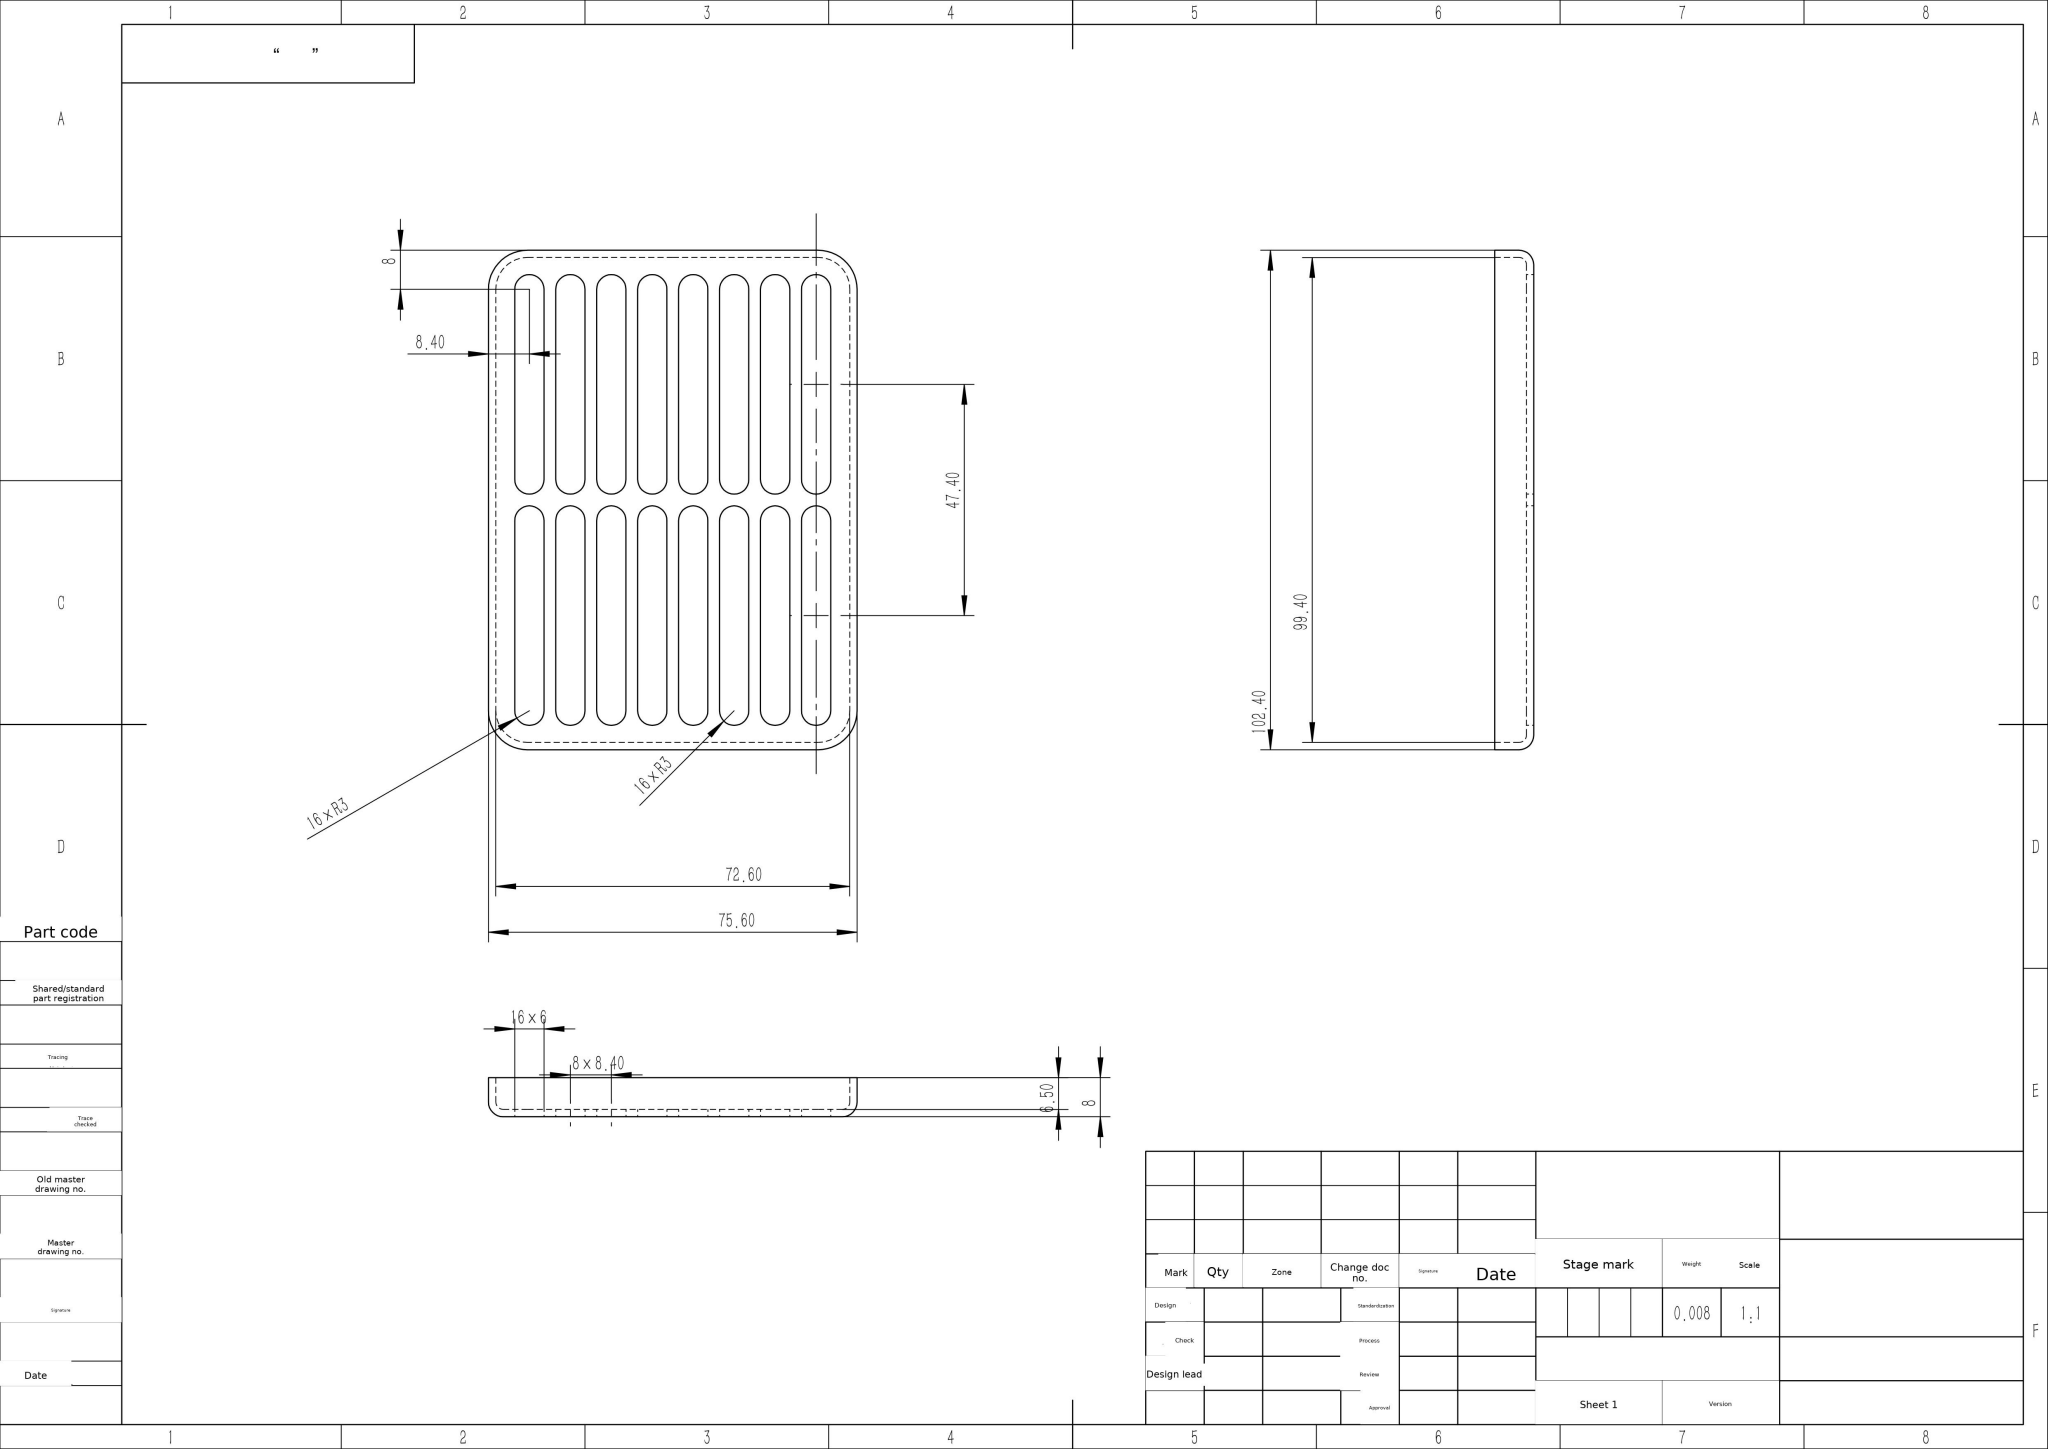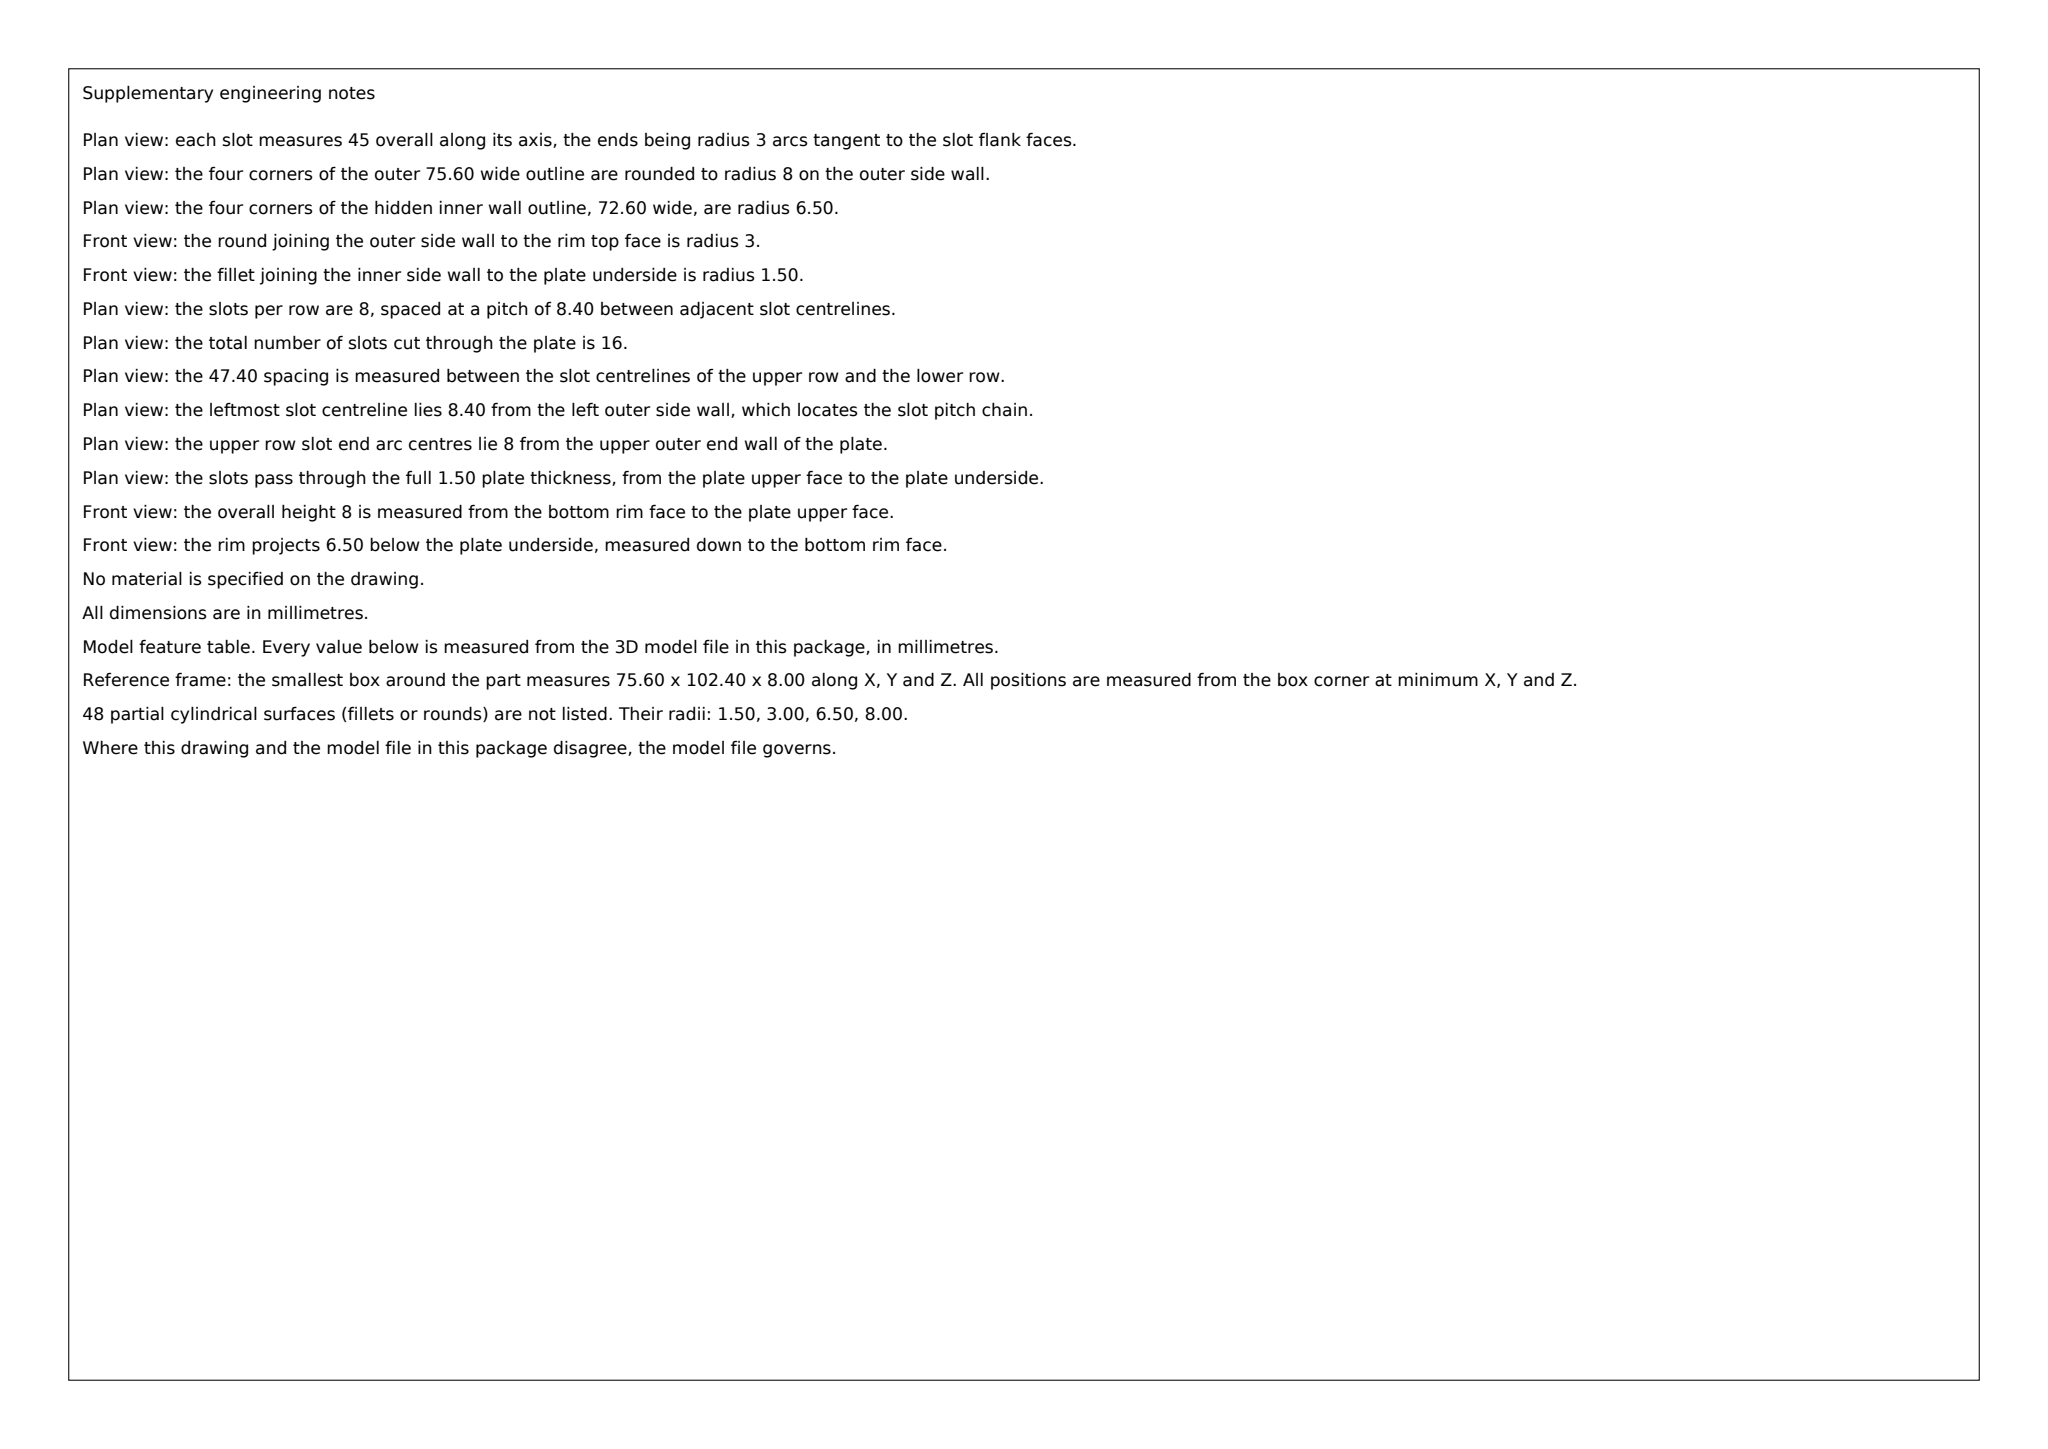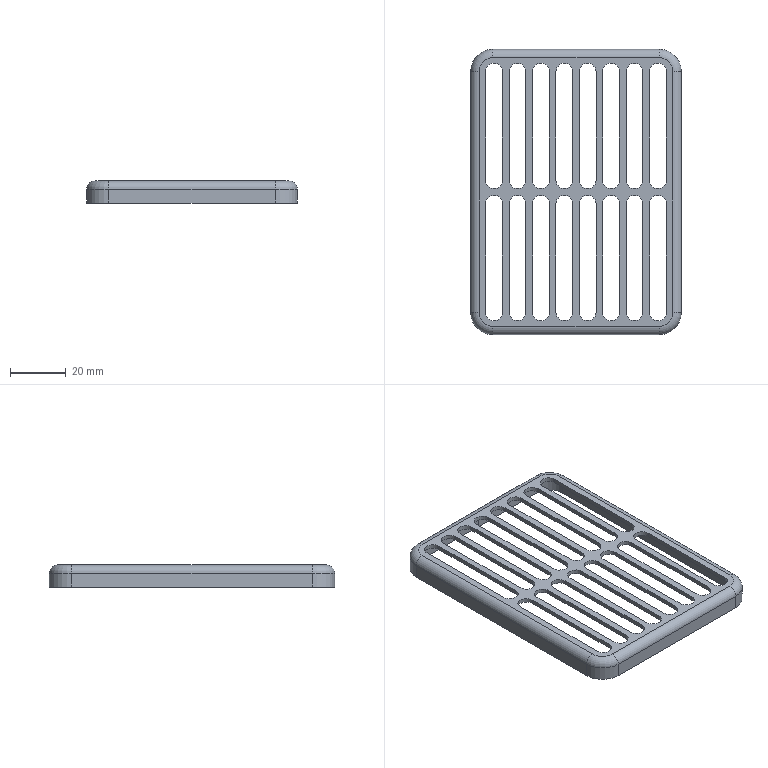Part | SolidWorks | mm | 1 solid | 110 faces | box 75.6 x 102.4 x 8 mm | volume 8033 mm3 | plane 53 | cylinder 49 | torus 8 | commonest cylinder face diameters 6 x36 3 x5 16 x4 13 x4